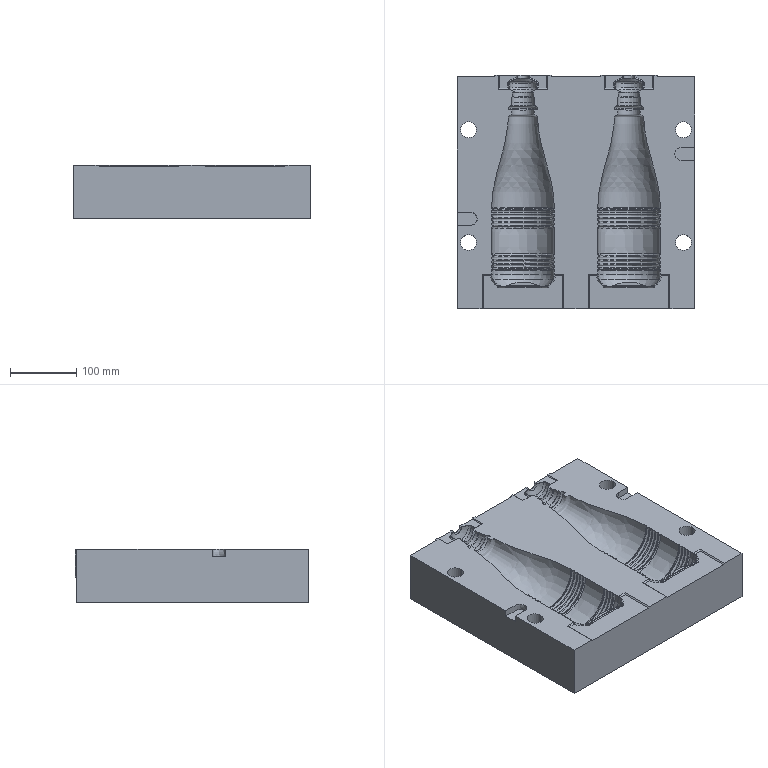CAM job | NX | mm | 3-axis | 1 set-up | 4 operations | part box 358 x 352.42 x 80.01
set-up 1
1. Cavity Milling | Mill Mill5 D29R5 | CAVITY_MILLING_1 | path 127688.548 mm | 49.97 min
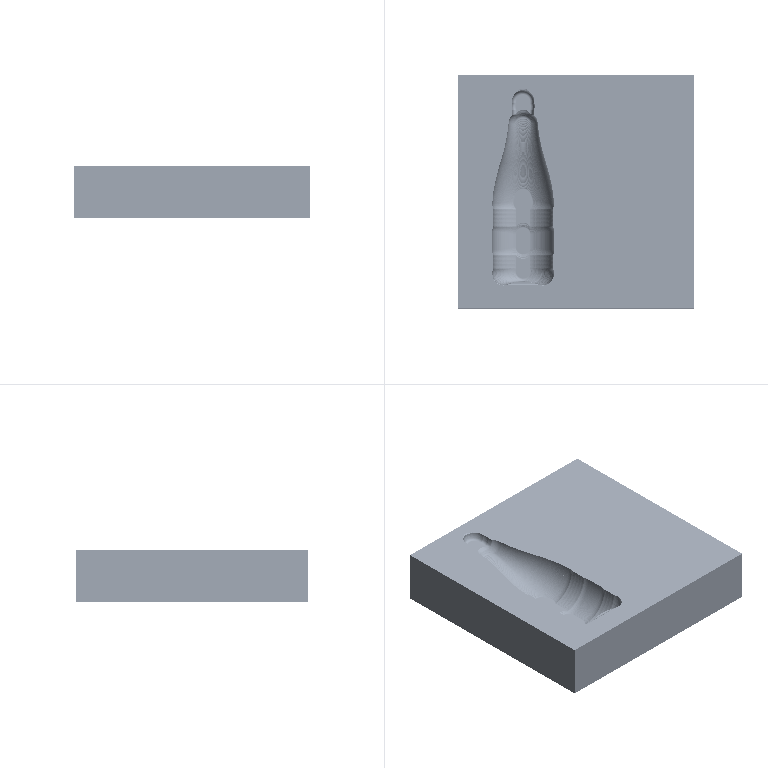2. Cavity Milling | Mill Mill5 D8 | CAVITY_MILL_1_COPY | path 25232.849 mm | 9.817 min
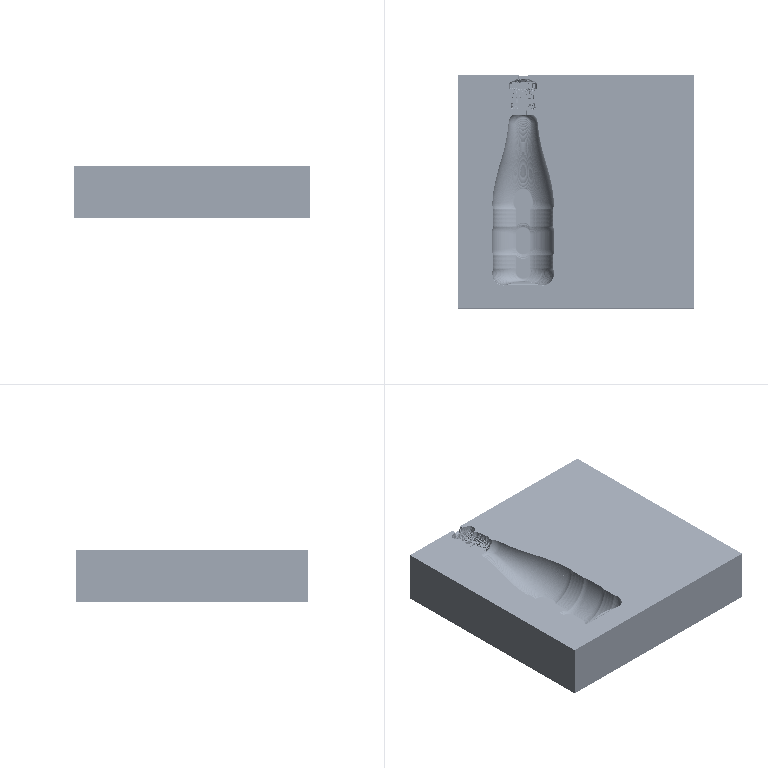3. Cavity Milling | Mill Mill5 D8 | CAVITY_MILL_1 | path 33430.643 mm | 12.35 min
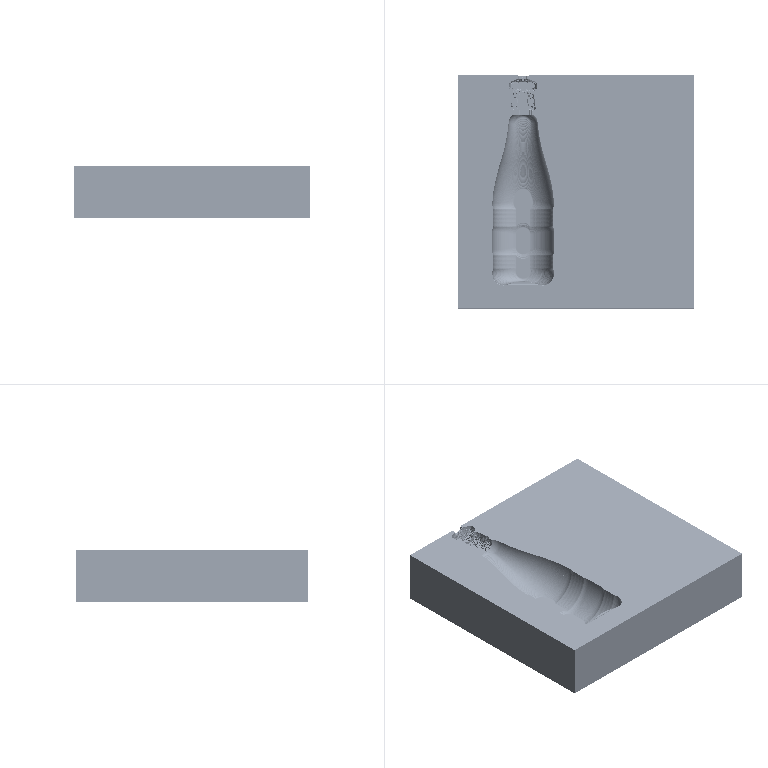4. Cavity Milling | Mill Mill5 D25R5 | CAVITY_MILLING_4 | path 164040.652 mm | 64.451 min